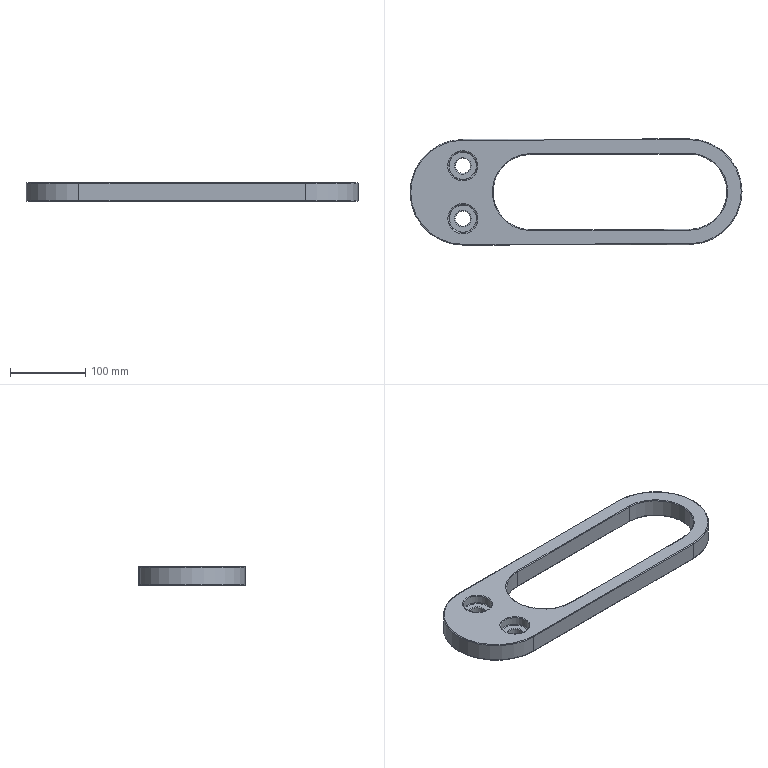Component | NX | A_PART_1 | 1 solid | 38 faces | volume 676499 mm3 | cylinder 16 | torus 14 | plane 8 | commonest cylinder face diameters 2 x8 100 x2 140 x2 38 x2 20 x2